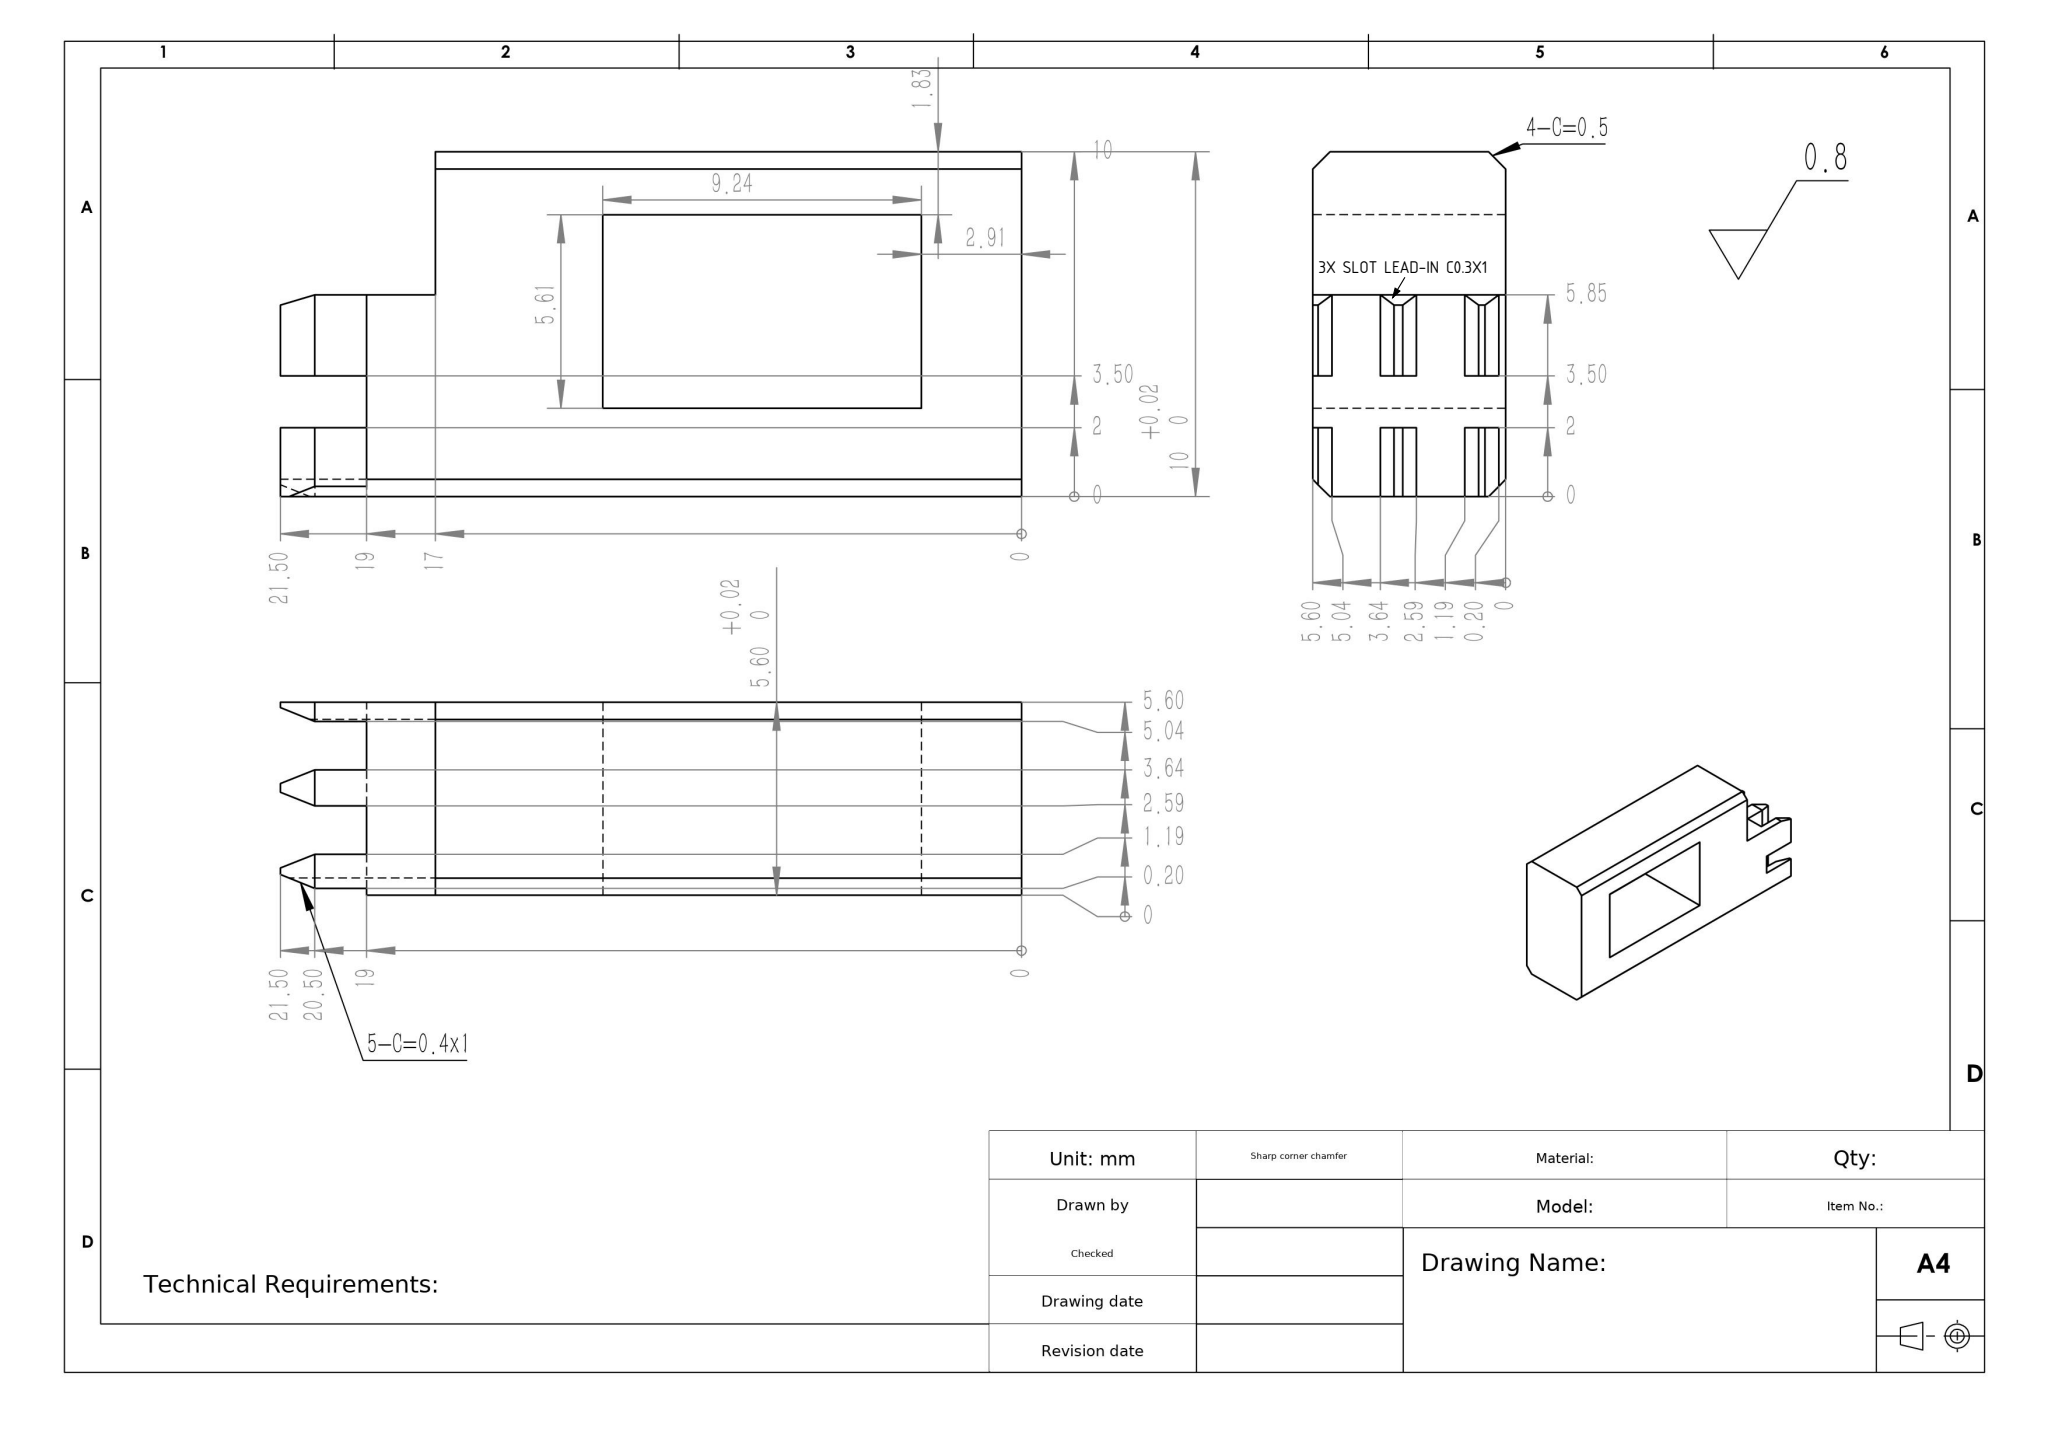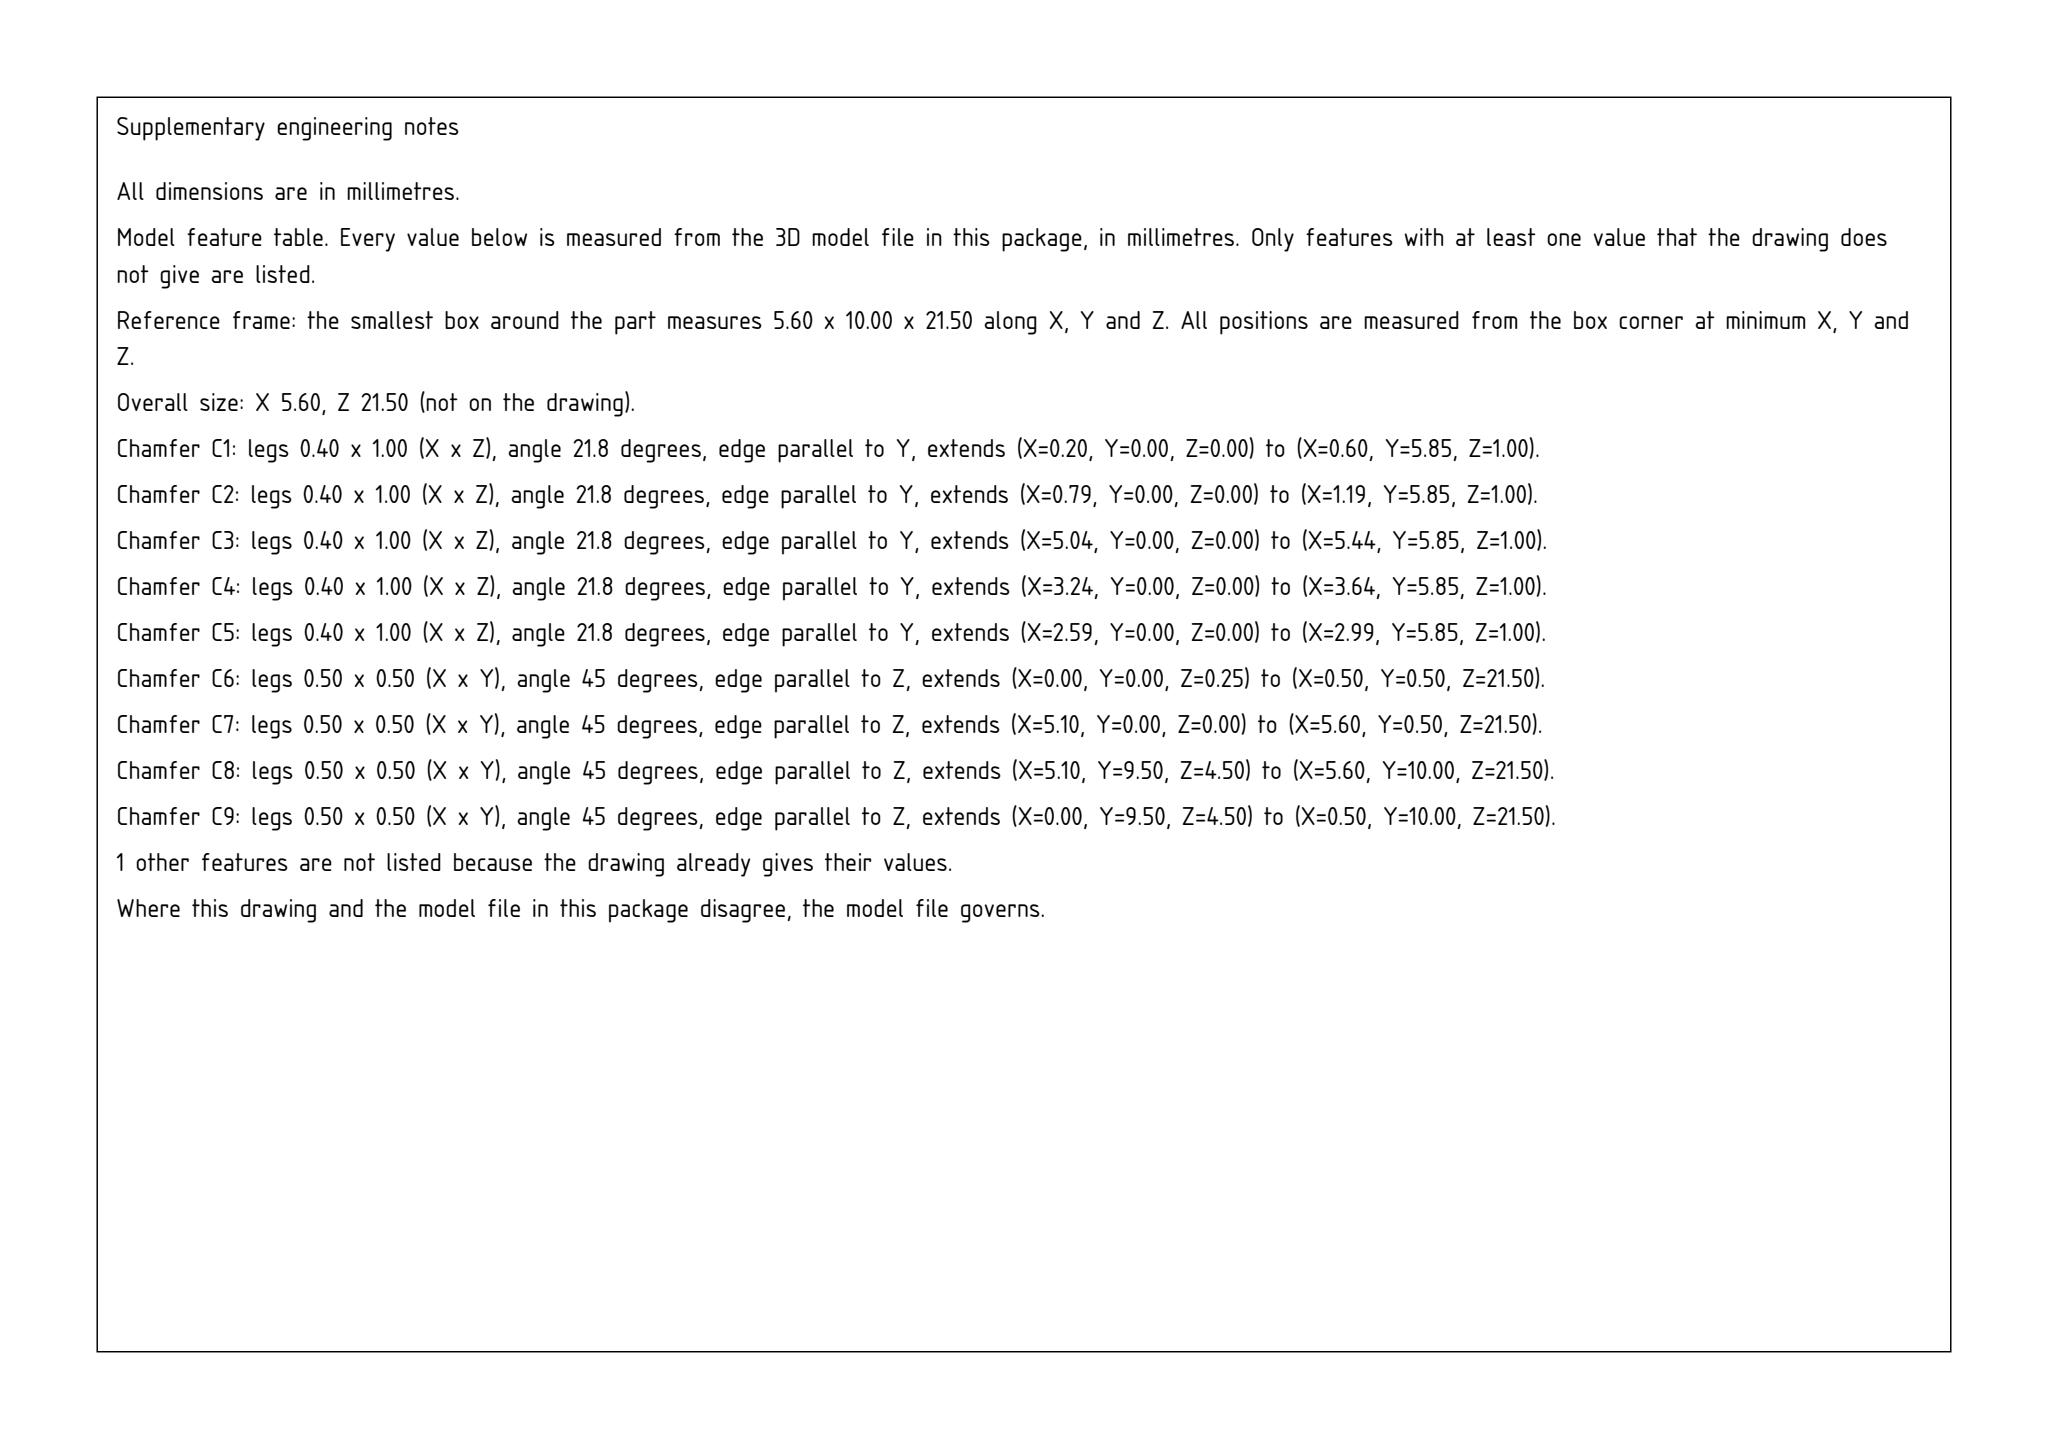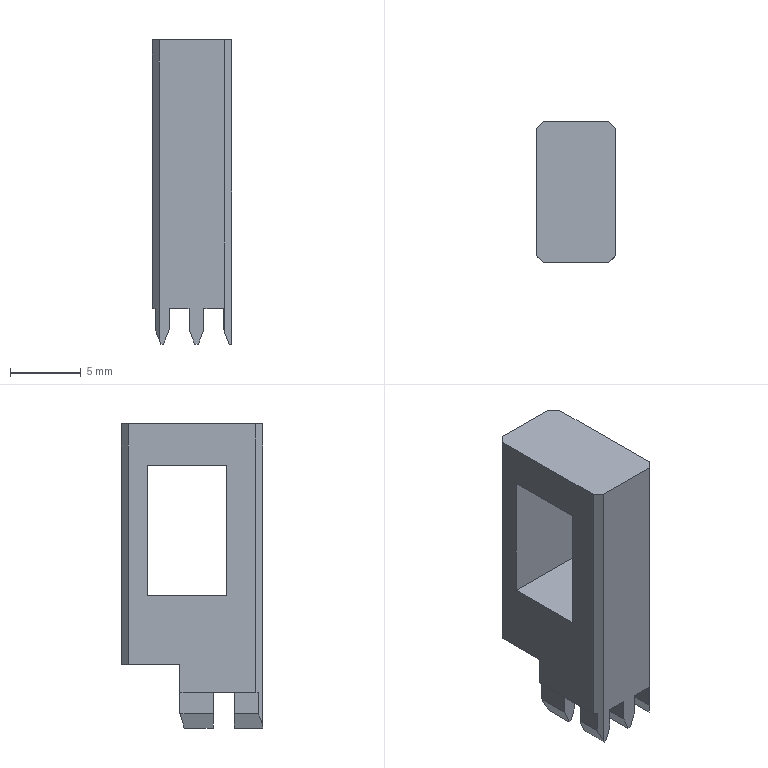Part | SolidWorks | mm | material 1.119 (C45G) | 1 solid | 51 faces | box 5.6 x 10 x 21.5 mm | volume 741 mm3 | plane 51
Drawing notes:
3X SLOT TOP LEAD-IN C0.3X1 (16.7 DEG) AT 5.80 FACE, FROM 0 END | from the solid: inclined_planes angle_to_xyz [90,16.7,73.3], bbox_from [0.2,5.5,0],[2.6,5.5,0],[5.0,5.5,0], size y=0.3 z=1.0; ramps to y=5.8 face (z 1.0-4.5) starting at z=0 end face
build123d program:
from build123d import *
from OCP.BRepFilletAPI import BRepFilletAPI_MakeChamfer

# Parameters (mm, degrees)
SKETCH1_W           = 5.6
SKETCH1_H           = 10
BOSS_EXTRUDE1_DEPTH = 21.5
SKETCH2_W           = 5.6
SKETCH2_H           = 4.15
CUT_EXTRUDE1_DEPTH  = 2.5
CHAMFER1_SIZE       = 0.5
SKETCH4_W           = 1.4
SKETCH4_H           = 5.85
SKETCH4_W_2         = 0.2
CUT_EXTRUDE2_DEPTH  = 2.5
CHAMFER2_SIZE       = 0.4
CHAMFER2_SIZE2      = 1
CUT_EXTRUDE3_DEPTH  = 25.364
CUT_EXTRUDE5_START  = -2.5
SKETCH7_W           = 8.413
SKETCH7_H           = 1.5
CUT_EXTRUDE5_DEPTH  = 2.5
SKETCH8_W           = 6.804
SKETCH8_H           = 4.15
CUT_EXTRUDE6_DEPTH  = 2
SKETCH9_W           = 9.238
SKETCH9_H           = 5.614
CUT_EXTRUDE7_DEPTH  = 10


with BuildPart() as part:
    # Sketch1 → Boss-Extrude1 (new body)
    with BuildSketch(Plane.XY):
        with Locations((2.8, 5)):
            Rectangle(SKETCH1_W, SKETCH1_H)
    extrude(amount=BOSS_EXTRUDE1_DEPTH)

    # Sketch2 → Cut-Extrude1 (cut)
    with BuildSketch(Plane(origin=(0, 0, 0), x_dir=(-1, 0, 0), z_dir=(0, 0, -1))):
        with Locations((-2.8, 7.925)):
            Rectangle(SKETCH2_W, SKETCH2_H)
    extrude(amount=-CUT_EXTRUDE1_DEPTH, mode=Mode.SUBTRACT)

    # Chamfer1
    chamfer1_edges = [part.edges().sort_by_distance(p)[0] for p in [
        (0, 10, 12),
        (5.6, 10, 12),
        (5.6, 0, 10.75),
        (0, 0, 10.75),
    ]]
    chamfer(chamfer1_edges, length=CHAMFER1_SIZE)

    # Sketch4 → Cut-Extrude2 (cut)
    with BuildSketch(Plane(origin=(0, 0, 0), x_dir=(-1, 0, 0), z_dir=(0, 0, -1))):
        with Locations((-1.89, 2.925)):
            Rectangle(SKETCH4_W, SKETCH4_H)
        with Locations((-4.34, 2.925)):
            Rectangle(SKETCH4_W, SKETCH4_H)
        with Locations((-0.1, 2.925)):
            Rectangle(SKETCH4_W_2, SKETCH4_H)
    extrude(amount=-CUT_EXTRUDE2_DEPTH, mode=Mode.SUBTRACT)

    # Chamfer2: one chamfer whose edges measure the first distance from different faces: ONE call of the kernel's chamfer builder (chamfer() names one face for all edges)
    chamfer2_edges_1 = [part.edges().sort_by_distance(p)[0] for p in [
        (1.19, 2.925, 0),
        (0.2, 3.075, 0),
    ]]
    chamfer2_side_1 = [part.faces().sort_by_distance(p)[0] for p in [
        (0.6981, 2.947, 0),
    ]]
    chamfer2_edges_2 = [part.edges().sort_by_distance(p)[0] for p in [
        (5.04, 2.925, 0),
    ]]
    chamfer2_side_2 = [part.faces().sort_by_distance(p)[0] for p in [
        (5.316, 3.034, 0),
    ]]
    chamfer2_edges_3 = [part.edges().sort_by_distance(p)[0] for p in [
        (3.64, 2.925, 0),
        (2.59, 2.925, 0),
    ]]
    chamfer2_side_3 = [part.faces().sort_by_distance(p)[0] for p in [
        (3.115, 2.925, 0),
    ]]
    chamfer2 = BRepFilletAPI_MakeChamfer(part.part.solid().wrapped)
    for e in chamfer2_edges_1:
        chamfer2.Add(CHAMFER2_SIZE, CHAMFER2_SIZE2, e.wrapped, chamfer2_side_1[0].wrapped)  # the first distance lies on this face
    for e in chamfer2_edges_2:
        chamfer2.Add(CHAMFER2_SIZE, CHAMFER2_SIZE2, e.wrapped, chamfer2_side_2[0].wrapped)  # the first distance lies on this face
    for e in chamfer2_edges_3:
        chamfer2.Add(CHAMFER2_SIZE, CHAMFER2_SIZE2, e.wrapped, chamfer2_side_3[0].wrapped)  # the first distance lies on this face
    add(Compound.cast(chamfer2.Shape()), mode=Mode.REPLACE)

    # Sketch5 → Cut-Extrude3 (cut, through all)
    with BuildSketch(Plane(origin=(5.6, 0, 0), x_dir=(0, 0, -1), z_dir=(1, 0, 0))):
        Polygon((0, 5.85), (-1, 5.85), (0, 5.55), align=None)
    extrude(amount=-CUT_EXTRUDE3_DEPTH, mode=Mode.SUBTRACT)

    # Sketch7 → Cut-Extrude5 (cut)
    with BuildSketch(Plane(origin=(0, 0, 0), x_dir=(-1, 0, 0), z_dir=(0, 0, -1)).offset(CUT_EXTRUDE5_START)):
        with Locations((-2.674, 2.75)):
            Rectangle(SKETCH7_W, SKETCH7_H)
    extrude(amount=CUT_EXTRUDE5_DEPTH, mode=Mode.SUBTRACT)

    # Sketch8 → Cut-Extrude6 (cut)
    with BuildSketch(Plane(origin=(0, 0, 2.5), x_dir=(-1, 0, 0), z_dir=(0, 0, -1))):
        with Locations((-3.05, 7.925)):
            Rectangle(SKETCH8_W, SKETCH8_H)
    extrude(amount=-CUT_EXTRUDE6_DEPTH, mode=Mode.SUBTRACT)

    # Sketch9 → Cut-Extrude7 (cut)
    with BuildSketch(Plane(origin=(5.6, 0, 0), x_dir=(0, 0, -1), z_dir=(1, 0, 0))):
        with Locations((-13.974, 5.366)):
            Rectangle(SKETCH9_W, SKETCH9_H)
    extrude(amount=-CUT_EXTRUDE7_DEPTH, mode=Mode.SUBTRACT)


solid = part.part